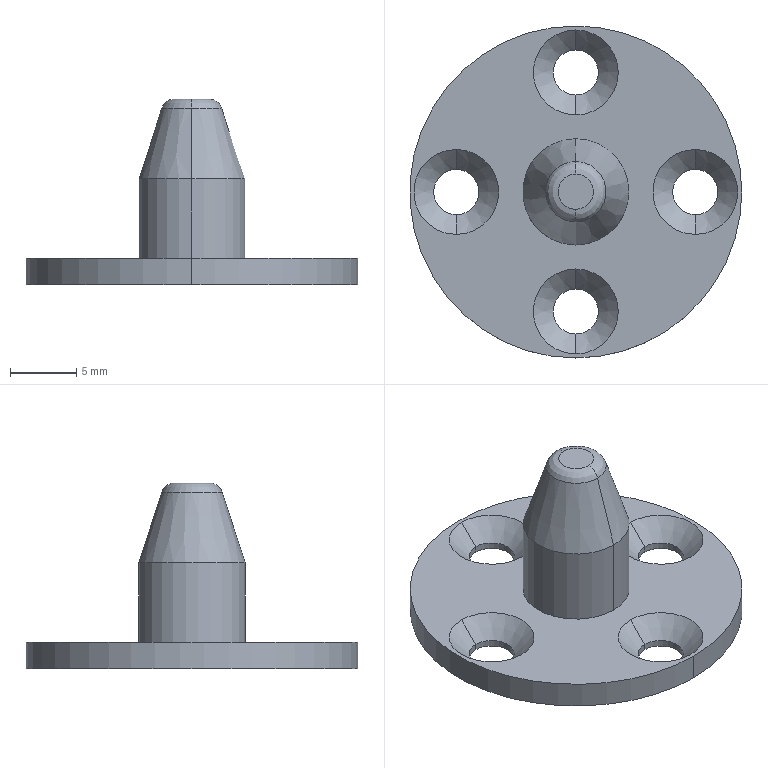CAM job | Mastercam | mm | 1 operations | part box 25 x 25 x 14
1. Drill/Counterbore | 7 - 4 倒角刀